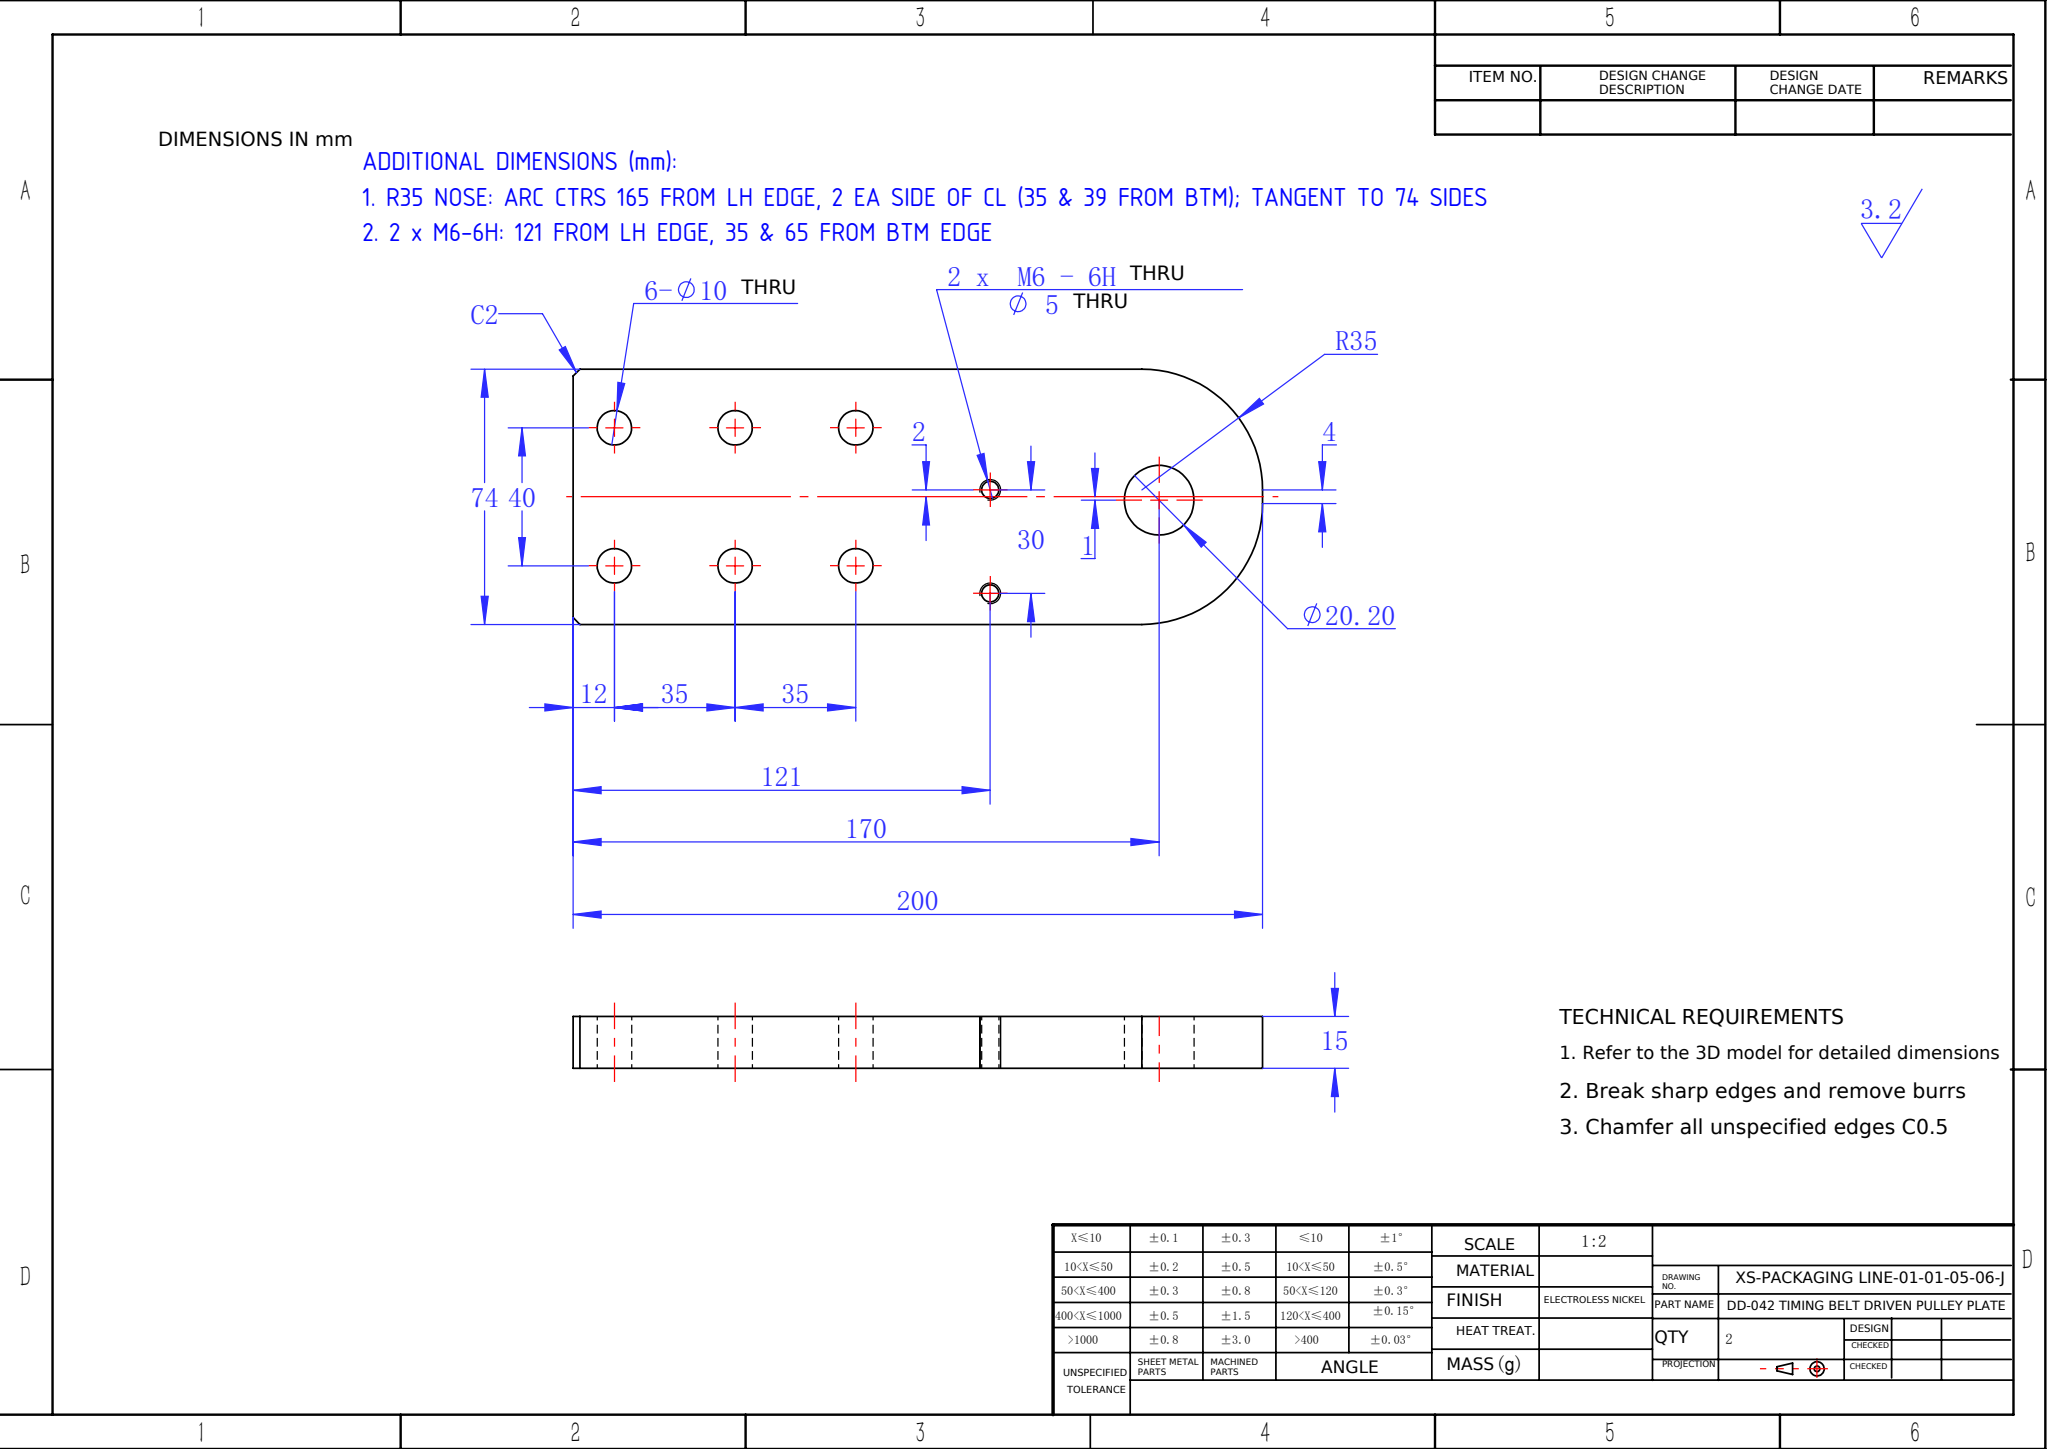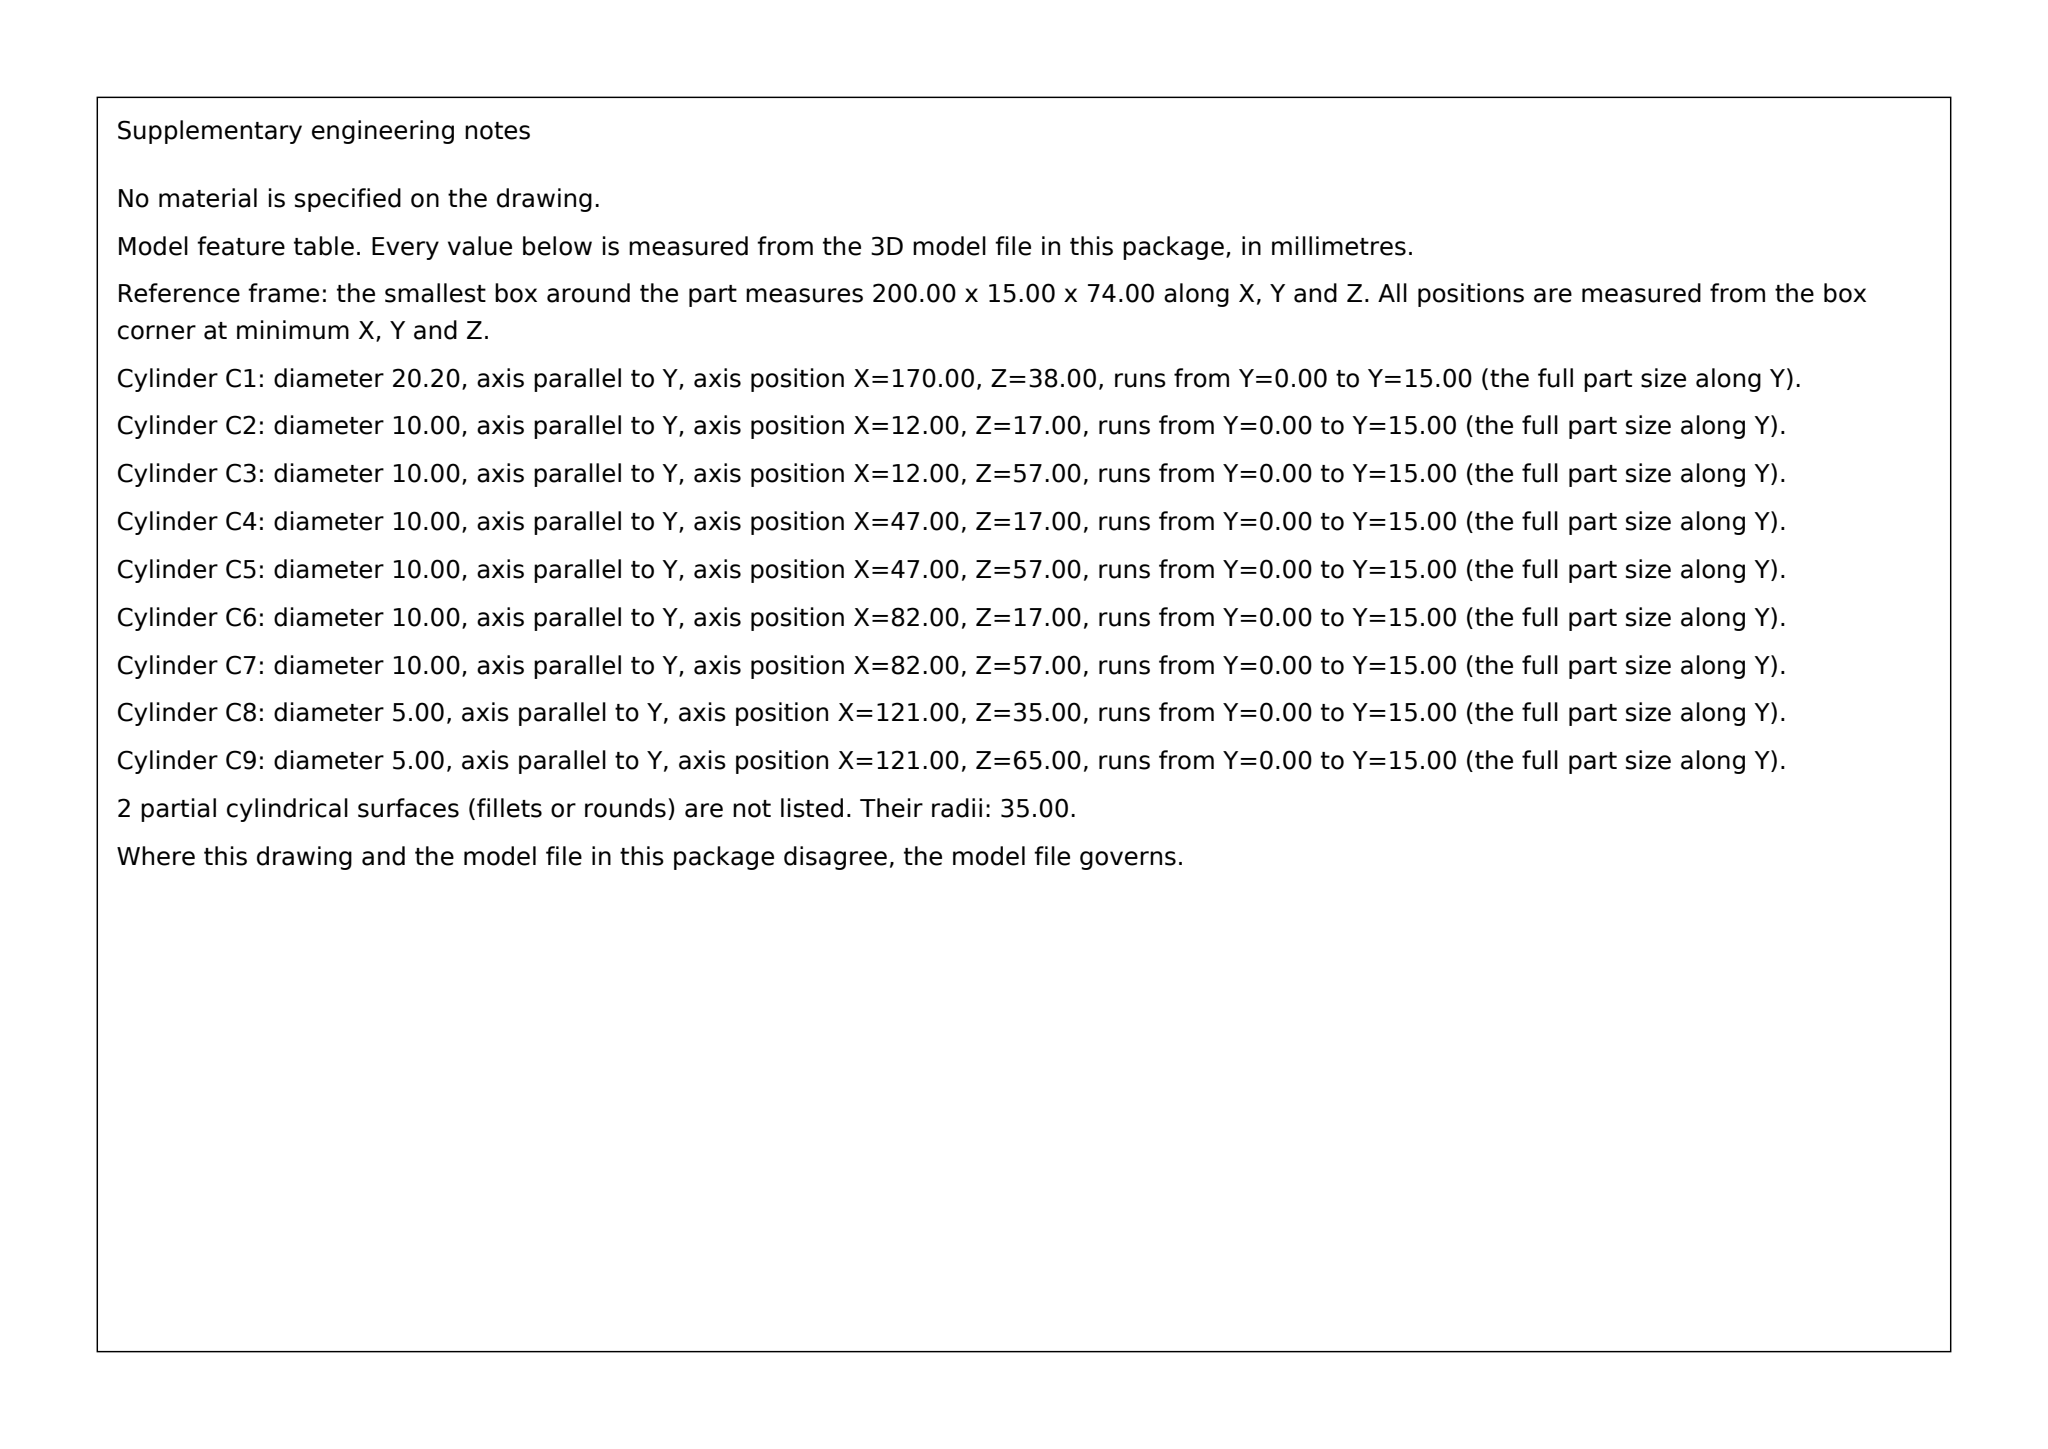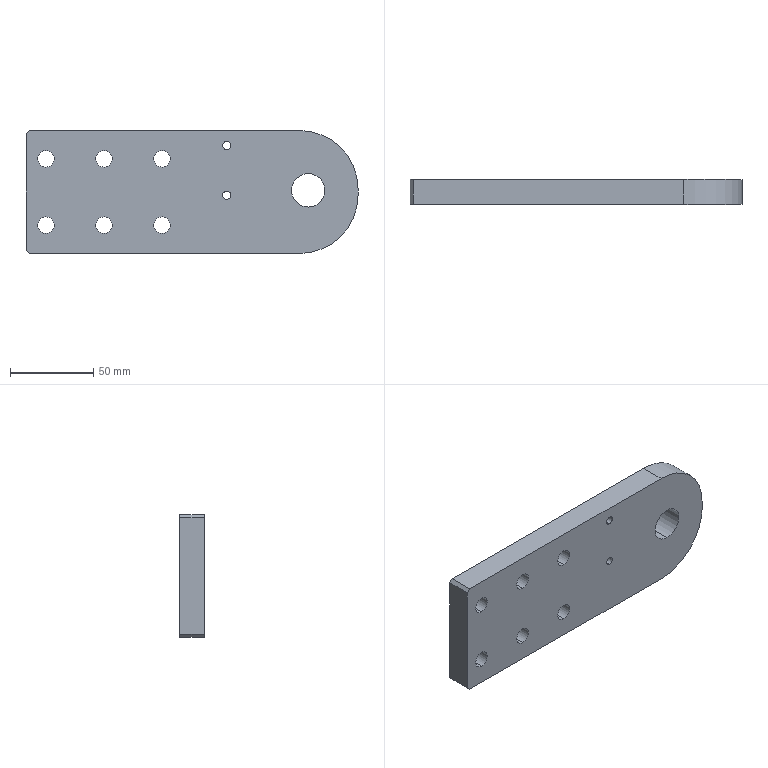Part | SolidWorks | mm | 1 solid | 28 faces | box 200 x 15 x 74 mm | volume 201589 mm3 | cylinder 20 | plane 8 | commonest cylinder face diameters 10 x12 5 x4 20.2 x2 70 x2
build123d program:
from build123d import *

# Parameters (mm, degrees)
SKETCH1_W           = 200
SKETCH1_H           = 74
BOSS_EXTRUDE1_DEPTH = 15
SKETCH2_R           = 10.1
CUT_EXTRUDE1_DEPTH  = 108.675
SKETCH4_R           = 5
CUT_EXTRUDE3_DEPTH  = 108.675
FILLET1_R           = 35
M6_TAPPED_HOLE1_D   = 5
CHAMFER1_SIZE       = 2


with BuildPart() as part:
    # Sketch1 → Boss-Extrude1 (new body)
    with BuildSketch(Plane(origin=(0, 0, 0), x_dir=(1, 0, 0), z_dir=(0, 1, 0))):
        Rectangle(SKETCH1_W, SKETCH1_H)
    extrude(amount=BOSS_EXTRUDE1_DEPTH)

    # Sketch2 → Cut-Extrude1 (cut, through all)
    with BuildSketch(Plane(origin=(0, 15, 0), x_dir=(1, 0, 0), z_dir=(0, 1, 0))):
        with Locations(Location((70, -1, 0), (0, 0, 270))):
            Circle(SKETCH2_R)
    extrude(amount=-CUT_EXTRUDE1_DEPTH, mode=Mode.SUBTRACT)

    # Sketch4 → Cut-Extrude3 (cut, through all)
    with BuildSketch(Plane.XZ):
        with Locations(Location((-88, 20, 0), (0, 0, 270))):
            Circle(SKETCH4_R)
        with Locations(Location((-53, 20, 0), (0, 0, 270))):
            Circle(SKETCH4_R)
        with Locations(Location((-18, 20, 0), (0, 0, 270))):
            Circle(SKETCH4_R)
        with Locations(Location((-88, -20, 0), (0, 0, 270))):
            Circle(SKETCH4_R)
        with Locations(Location((-53, -20, 0), (0, 0, 270))):
            Circle(SKETCH4_R)
        with Locations(Location((-18, -20, 0), (0, 0, 270))):
            Circle(SKETCH4_R)
    extrude(amount=-CUT_EXTRUDE3_DEPTH, mode=Mode.SUBTRACT)

    # Fillet1
    fillet1_edges = [part.edges().sort_by_distance(p)[0] for p in [
        (100, 7.5, -37),
        (100, 7.5, 37),
    ]]
    fillet(fillet1_edges, radius=FILLET1_R)

    # M6 Tapped Hole1 (through all)
    with Locations(Plane(origin=(0, 0, 0), x_dir=(-1, 0, 0), z_dir=(0, -1, 0))):
        with Locations((-21, -28), (-21, 2)):
            Hole(M6_TAPPED_HOLE1_D / 2)

    # Chamfer1
    chamfer1_edges = [part.edges().sort_by_distance(p)[0] for p in [
        (-100, 7.5, -37),
        (-100, 7.5, 37),
    ]]
    chamfer(chamfer1_edges, length=CHAMFER1_SIZE)


solid = part.part